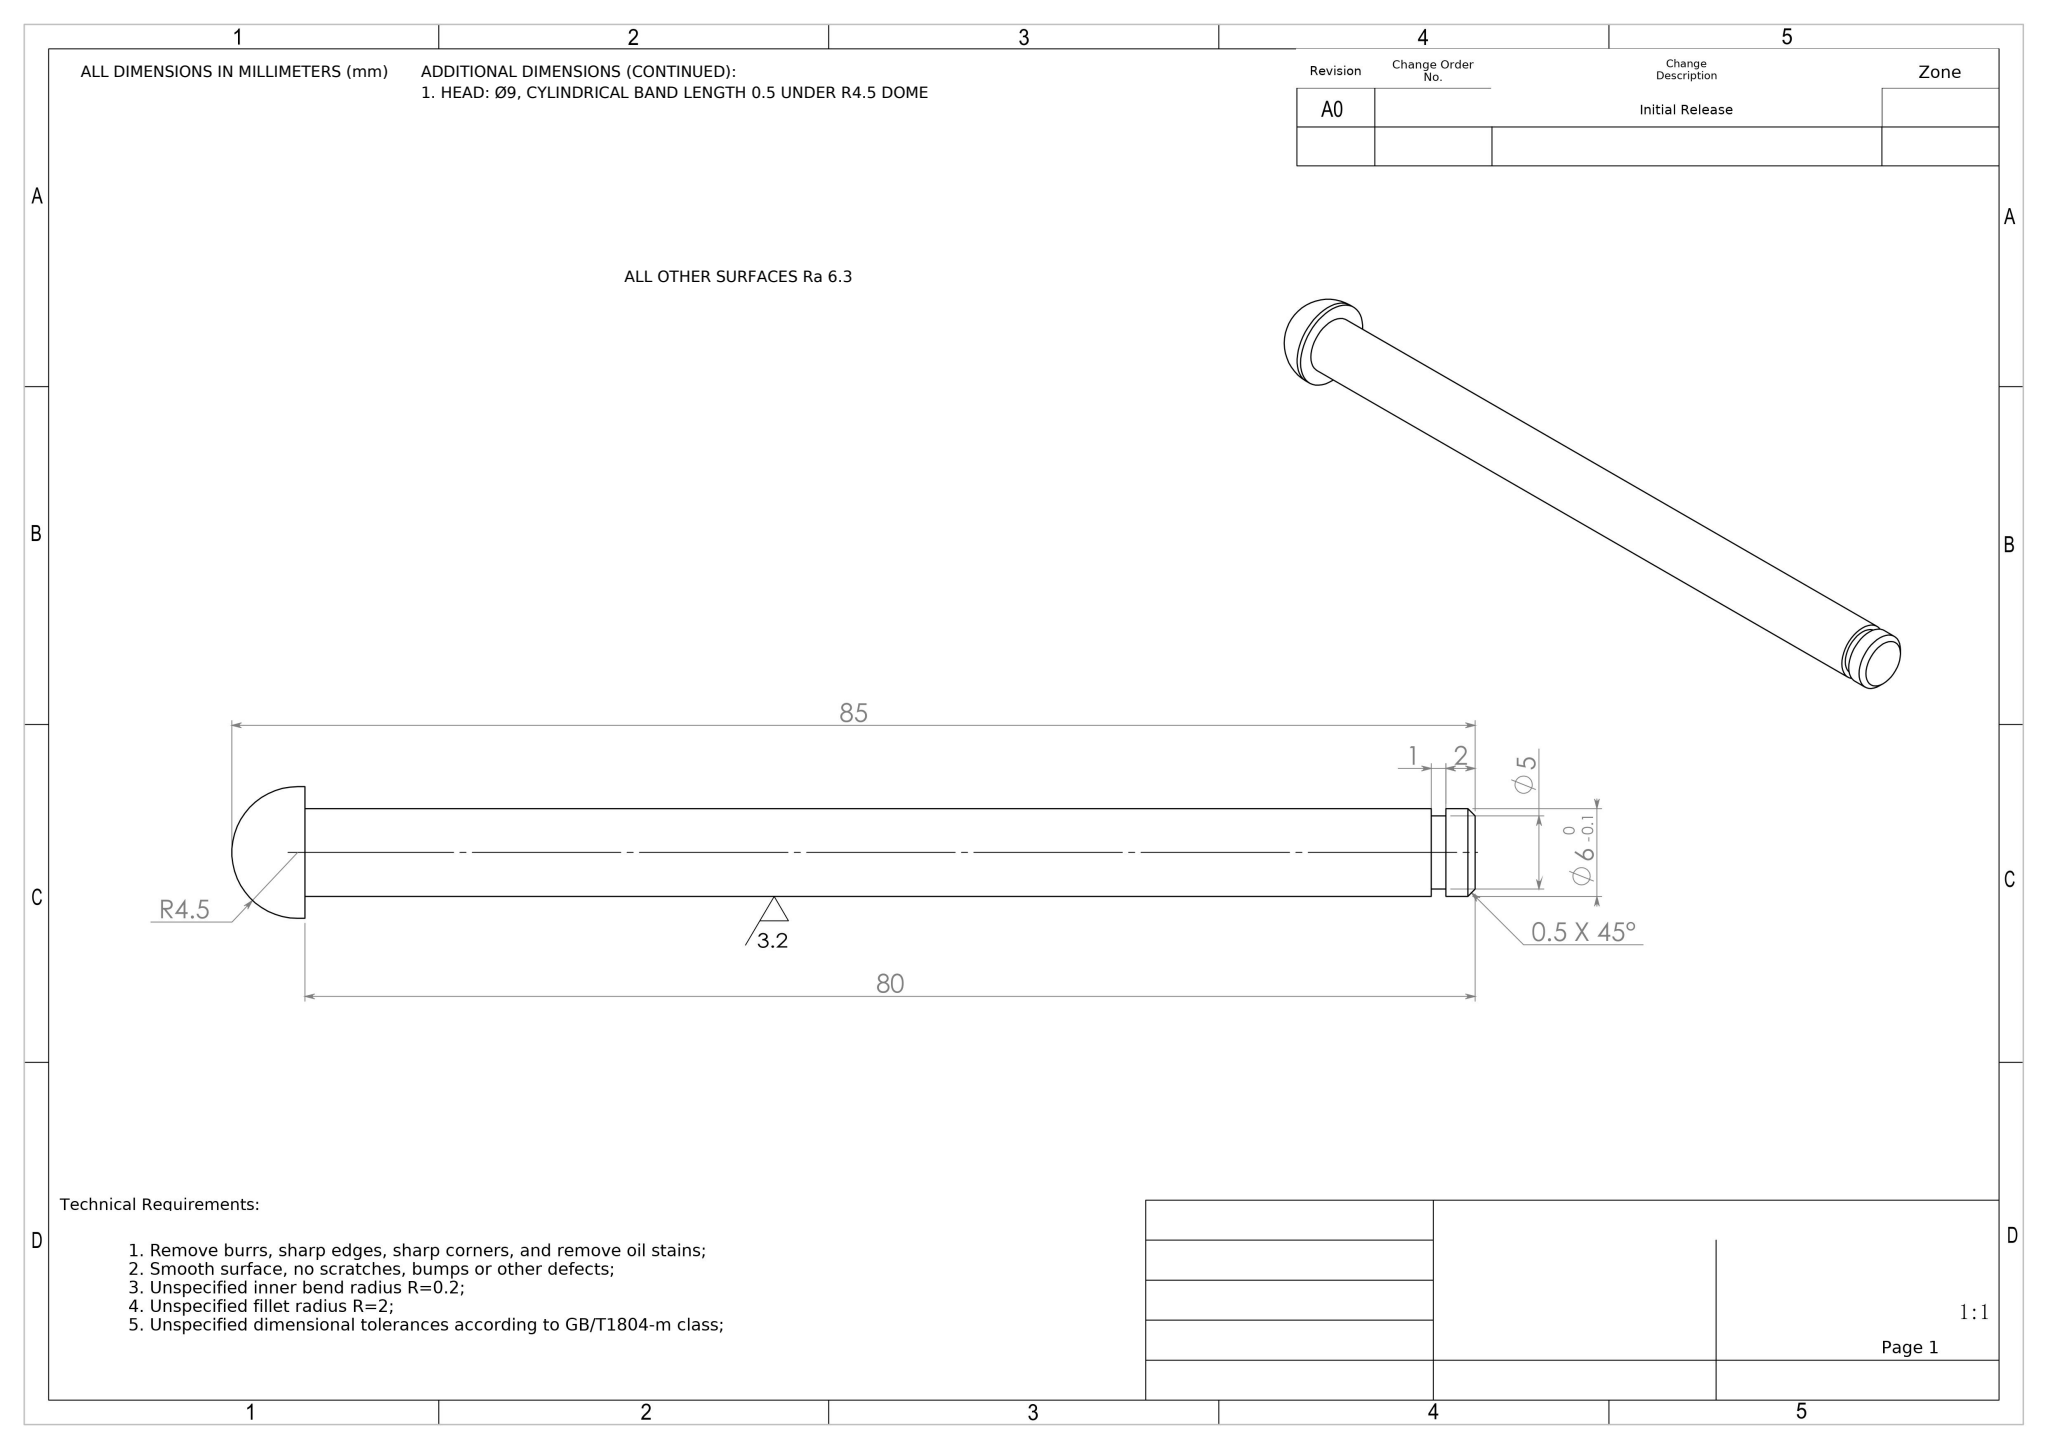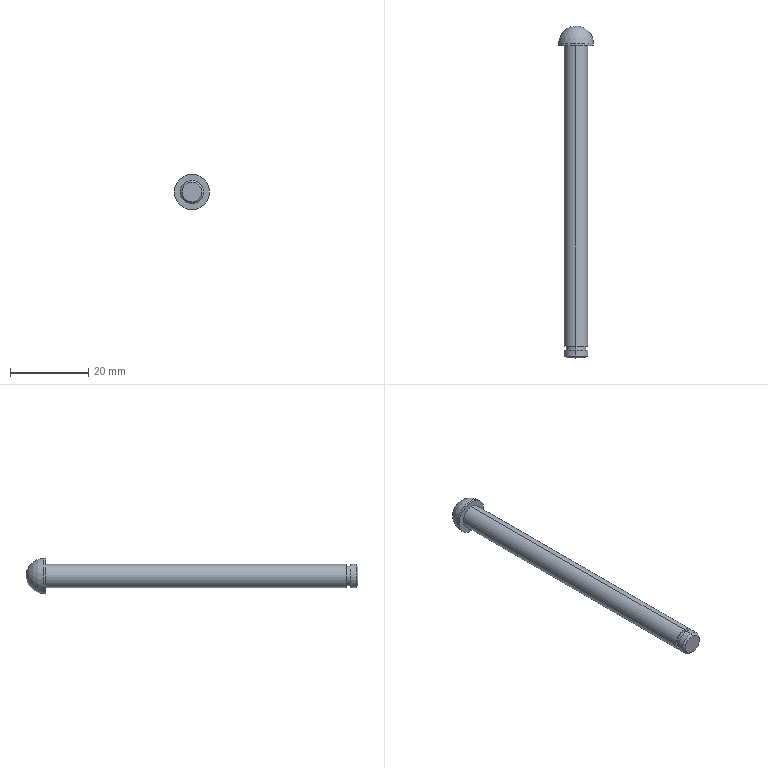Part | NX | mm | 1 solid | 15 faces | box 9 x 85 x 9 mm | volume 2474 mm3 | cylinder 8 | plane 4 | cone 2 | sphere 1 | commonest cylinder face diameters 6 x4 5 x2 9 x2
STEP:
#1=COLOUR_RGB('',0.7529,0.7529,0.7529);
#2=FILL_AREA_STYLE_COLOUR('',#1);
#3=FILL_AREA_STYLE('',(#2));
#4=SURFACE_STYLE_FILL_AREA(#3);
#5=SURFACE_SIDE_STYLE('',(#4));
#6=SURFACE_STYLE_USAGE(.BOTH.,#5);
#7=PRESENTATION_STYLE_ASSIGNMENT((#6));
#8=CARTESIAN_POINT('',(0.,2.,-3.));
#9=VERTEX_POINT('',#8);
#10=CARTESIAN_POINT('',(0.,2.,3.));
#11=VERTEX_POINT('',#10);
#12=CARTESIAN_POINT('',(0.,2.,0.));
#13=DIRECTION('',(0.,-1.,0.));
#14=DIRECTION('',(0.,0.,-1.));
#15=AXIS2_PLACEMENT_3D('',#12,#13,#14);
#16=CIRCLE('',#15,3.);
#17=EDGE_CURVE('',#9,#11,#16,.T.);
#18=ORIENTED_EDGE('',*,*,#17,.T.);
#19=CARTESIAN_POINT('',(0.,0.5,3.));
#20=VERTEX_POINT('',#19);
#21=CARTESIAN_POINT('',(0.,80.,3.));
#22=DIRECTION('',(0.,-1.,0.));
#23=VECTOR('',#22,1000.);
#24=LINE('',#21,#23);
#25=EDGE_CURVE('',#11,#20,#24,.T.);
#26=ORIENTED_EDGE('',*,*,#25,.T.);
#27=CARTESIAN_POINT('',(0.,0.5,-3.));
#28=VERTEX_POINT('',#27);
#29=CARTESIAN_POINT('',(0.,0.5,0.));
#30=DIRECTION('',(0.,1.,0.));
#31=DIRECTION('',(0.,0.,1.));
#32=AXIS2_PLACEMENT_3D('',#29,#30,#31);
#33=CIRCLE('',#32,3.);
#34=EDGE_CURVE('',#20,#28,#33,.T.);
#35=ORIENTED_EDGE('',*,*,#34,.T.);
#36=CARTESIAN_POINT('',(0.,80.,-3.));
#37=DIRECTION('',(0.,-1.,0.));
#38=VECTOR('',#37,1000.);
#39=LINE('',#36,#38);
#40=EDGE_CURVE('',#9,#28,#39,.T.);
#41=ORIENTED_EDGE('',*,*,#40,.F.);
#42=EDGE_LOOP('',(#18,#26,#35,#41));
#43=FACE_OUTER_BOUND('',#42,.T.);
#44=CARTESIAN_POINT('',(0.,80.,0.));
#45=DIRECTION('',(0.,-1.,0.));
#46=DIRECTION('',(0.,0.,-1.));
#47=AXIS2_PLACEMENT_3D('',#44,#45,#46);
#48=CYLINDRICAL_SURFACE('',#47,3.);
#49=ADVANCED_FACE('',(#43),#48,.T.);
#50=CARTESIAN_POINT('',(0.,0.,-2.5));
#51=VERTEX_POINT('',#50);
#52=CARTESIAN_POINT('',(0.,0.,2.5));
#53=VERTEX_POINT('',#52);
#54=CARTESIAN_POINT('',(0.,0.,0.));
#55=DIRECTION('',(0.,-1.,0.));
#56=DIRECTION('',(0.,0.,1.));
#57=AXIS2_PLACEMENT_3D('',#54,#55,#56);
#58=CIRCLE('',#57,2.5);
#59=EDGE_CURVE('',#51,#53,#58,.T.);
#60=ORIENTED_EDGE('',*,*,#59,.F.);
#61=CARTESIAN_POINT('',(0.,0.5,-3.));
#62=DIRECTION('',(0.,0.7071,-0.7071));
#63=VECTOR('',#62,1000.);
#64=LINE('',#61,#63);
#65=EDGE_CURVE('',#51,#28,#64,.T.);
#66=ORIENTED_EDGE('',*,*,#65,.T.);
#67=ORIENTED_EDGE('',*,*,#34,.F.);
#68=CARTESIAN_POINT('',(0.,0.5,3.));
#69=DIRECTION('',(0.,0.7071,0.7071));
#70=VECTOR('',#69,1000.);
#71=LINE('',#68,#70);
#72=EDGE_CURVE('',#53,#20,#71,.T.);
#73=ORIENTED_EDGE('',*,*,#72,.F.);
#74=EDGE_LOOP('',(#60,#66,#67,#73));
#75=FACE_OUTER_BOUND('',#74,.T.);
#76=CARTESIAN_POINT('',(0.,0.5,0.));
#77=DIRECTION('',(0.,1.,0.));
#78=DIRECTION('',(0.,0.,1.));
#79=AXIS2_PLACEMENT_3D('',#76,#77,#78);
#80=CONICAL_SURFACE('',#79,3.,0.7854);
#81=ADVANCED_FACE('',(#75),#80,.T.);
#82=CARTESIAN_POINT('',(0.,3.,-2.5));
#83=VERTEX_POINT('',#82);
#84=CARTESIAN_POINT('',(0.,3.,2.5));
#85=VERTEX_POINT('',#84);
#86=CARTESIAN_POINT('',(0.,3.,0.));
#87=DIRECTION('',(0.,-1.,0.));
#88=DIRECTION('',(0.,0.,-1.));
#89=AXIS2_PLACEMENT_3D('',#86,#87,#88);
#90=CIRCLE('',#89,2.5);
#91=EDGE_CURVE('',#83,#85,#90,.T.);
#92=ORIENTED_EDGE('',*,*,#91,.T.);
#93=CARTESIAN_POINT('',(0.,2.,2.5));
#94=VERTEX_POINT('',#93);
#95=CARTESIAN_POINT('',(0.,0.,2.5));
#96=DIRECTION('',(0.,-1.,0.));
#97=VECTOR('',#96,1000.);
#98=LINE('',#95,#97);
#99=EDGE_CURVE('',#85,#94,#98,.T.);
#100=ORIENTED_EDGE('',*,*,#99,.T.);
#101=CARTESIAN_POINT('',(0.,2.,-2.5));
#102=VERTEX_POINT('',#101);
#103=CARTESIAN_POINT('',(0.,2.,0.));
#104=DIRECTION('',(0.,-1.,0.));
#105=DIRECTION('',(0.,0.,-1.));
#106=AXIS2_PLACEMENT_3D('',#103,#104,#105);
#107=CIRCLE('',#106,2.5);
#108=EDGE_CURVE('',#102,#94,#107,.T.);
#109=ORIENTED_EDGE('',*,*,#108,.F.);
#110=CARTESIAN_POINT('',(0.,0.,-2.5));
#111=DIRECTION('',(0.,-1.,0.));
#112=VECTOR('',#111,1000.);
#113=LINE('',#110,#112);
#114=EDGE_CURVE('',#83,#102,#113,.T.);
#115=ORIENTED_EDGE('',*,*,#114,.F.);
#116=EDGE_LOOP('',(#92,#100,#109,#115));
#117=FACE_OUTER_BOUND('',#116,.T.);
#118=CARTESIAN_POINT('',(0.,0.,0.));
#119=DIRECTION('',(0.,-1.,0.));
#120=DIRECTION('',(0.,0.,-1.));
#121=AXIS2_PLACEMENT_3D('',#118,#119,#120);
#122=CYLINDRICAL_SURFACE('',#121,2.5);
#123=ADVANCED_FACE('',(#117),#122,.T.);
#124=CARTESIAN_POINT('',(0.,80.5,-4.5));
#125=VERTEX_POINT('',#124);
#126=CARTESIAN_POINT('',(0.,80.5,4.5));
#127=VERTEX_POINT('',#126);
#128=CARTESIAN_POINT('',(0.,80.5,0.));
#129=DIRECTION('',(0.,-1.,0.));
#130=DIRECTION('',(0.,0.,-1.));
#131=AXIS2_PLACEMENT_3D('',#128,#129,#130);
#132=CIRCLE('',#131,4.5);
#133=EDGE_CURVE('',#125,#127,#132,.T.);
#134=ORIENTED_EDGE('',*,*,#133,.T.);
#135=CARTESIAN_POINT('',(0.,80.,4.5));
#136=VERTEX_POINT('',#135);
#137=CARTESIAN_POINT('',(0.,85.,4.5));
#138=DIRECTION('',(0.,-1.,0.));
#139=VECTOR('',#138,1000.);
#140=LINE('',#137,#139);
#141=EDGE_CURVE('',#127,#136,#140,.T.);
#142=ORIENTED_EDGE('',*,*,#141,.T.);
#143=CARTESIAN_POINT('',(0.,80.,-4.5));
#144=VERTEX_POINT('',#143);
#145=CARTESIAN_POINT('',(0.,80.,0.));
#146=DIRECTION('',(0.,1.,0.));
#147=DIRECTION('',(0.,0.,1.));
#148=AXIS2_PLACEMENT_3D('',#145,#146,#147);
#149=CIRCLE('',#148,4.5);
#150=EDGE_CURVE('',#136,#144,#149,.T.);
#151=ORIENTED_EDGE('',*,*,#150,.T.);
#152=CARTESIAN_POINT('',(0.,85.,-4.5));
#153=DIRECTION('',(0.,-1.,0.));
#154=VECTOR('',#153,1000.);
#155=LINE('',#152,#154);
#156=EDGE_CURVE('',#125,#144,#155,.T.);
#157=ORIENTED_EDGE('',*,*,#156,.F.);
#158=EDGE_LOOP('',(#134,#142,#151,#157));
#159=FACE_OUTER_BOUND('',#158,.T.);
#160=CARTESIAN_POINT('',(0.,85.,0.));
#161=DIRECTION('',(0.,-1.,0.));
#162=DIRECTION('',(0.,0.,-1.));
#163=AXIS2_PLACEMENT_3D('',#160,#161,#162);
#164=CYLINDRICAL_SURFACE('',#163,4.5);
#165=ADVANCED_FACE('',(#159),#164,.T.);
#166=CARTESIAN_POINT('',(0.,80.,3.));
#167=VERTEX_POINT('',#166);
#168=CARTESIAN_POINT('',(0.,80.,-3.));
#169=VERTEX_POINT('',#168);
#170=CARTESIAN_POINT('',(0.,80.,0.));
#171=DIRECTION('',(0.,1.,0.));
#172=DIRECTION('',(0.,0.,1.));
#173=AXIS2_PLACEMENT_3D('',#170,#171,#172);
#174=CIRCLE('',#173,3.);
#175=EDGE_CURVE('',#167,#169,#174,.T.);
#176=ORIENTED_EDGE('',*,*,#175,.F.);
#177=CARTESIAN_POINT('',(0.,3.,3.));
#178=VERTEX_POINT('',#177);
#179=CARTESIAN_POINT('',(0.,80.,3.));
#180=DIRECTION('',(0.,-1.,0.));
#181=VECTOR('',#180,1000.);
#182=LINE('',#179,#181);
#183=EDGE_CURVE('',#167,#178,#182,.T.);
#184=ORIENTED_EDGE('',*,*,#183,.T.);
#185=CARTESIAN_POINT('',(0.,3.,-3.));
#186=VERTEX_POINT('',#185);
#187=CARTESIAN_POINT('',(0.,3.,0.));
#188=DIRECTION('',(0.,-1.,0.));
#189=DIRECTION('',(0.,0.,-1.));
#190=AXIS2_PLACEMENT_3D('',#187,#188,#189);
#191=CIRCLE('',#190,3.);
#192=EDGE_CURVE('',#186,#178,#191,.T.);
#193=ORIENTED_EDGE('',*,*,#192,.F.);
#194=CARTESIAN_POINT('',(0.,80.,-3.));
#195=DIRECTION('',(0.,-1.,0.));
#196=VECTOR('',#195,1000.);
#197=LINE('',#194,#196);
#198=EDGE_CURVE('',#169,#186,#197,.T.);
#199=ORIENTED_EDGE('',*,*,#198,.F.);
#200=EDGE_LOOP('',(#176,#184,#193,#199));
#201=FACE_OUTER_BOUND('',#200,.T.);
#202=CARTESIAN_POINT('',(0.,80.,0.));
#203=DIRECTION('',(0.,-1.,0.));
#204=DIRECTION('',(0.,0.,-1.));
#205=AXIS2_PLACEMENT_3D('',#202,#203,#204);
#206=CYLINDRICAL_SURFACE('',#205,3.);
#207=ADVANCED_FACE('',(#201),#206,.T.);
#208=ORIENTED_EDGE('',*,*,#183,.F.);
#209=CARTESIAN_POINT('',(0.,80.,0.));
#210=DIRECTION('',(0.,1.,0.));
#211=DIRECTION('',(0.,0.,1.));
#212=AXIS2_PLACEMENT_3D('',#209,#210,#211);
#213=CIRCLE('',#212,3.);
#214=EDGE_CURVE('',#169,#167,#213,.T.);
#215=ORIENTED_EDGE('',*,*,#214,.F.);
#216=ORIENTED_EDGE('',*,*,#198,.T.);
#217=CARTESIAN_POINT('',(0.,3.,0.));
#218=DIRECTION('',(0.,-1.,0.));
#219=DIRECTION('',(0.,0.,-1.));
#220=AXIS2_PLACEMENT_3D('',#217,#218,#219);
#221=CIRCLE('',#220,3.);
#222=EDGE_CURVE('',#178,#186,#221,.T.);
#223=ORIENTED_EDGE('',*,*,#222,.F.);
#224=EDGE_LOOP('',(#208,#215,#216,#223));
#225=FACE_OUTER_BOUND('',#224,.T.);
#226=CARTESIAN_POINT('',(0.,80.,0.));
#227=DIRECTION('',(0.,-1.,0.));
#228=DIRECTION('',(0.,0.,-1.));
#229=AXIS2_PLACEMENT_3D('',#226,#227,#228);
#230=CYLINDRICAL_SURFACE('',#229,3.);
#231=ADVANCED_FACE('',(#225),#230,.T.);
#232=CARTESIAN_POINT('',(0.,80.,0.));
#233=DIRECTION('',(0.,1.,0.));
#234=DIRECTION('',(0.,0.,1.));
#235=AXIS2_PLACEMENT_3D('',#232,#233,#234);
#236=CIRCLE('',#235,4.5);
#237=EDGE_CURVE('',#144,#136,#236,.T.);
#238=ORIENTED_EDGE('',*,*,#237,.F.);
#239=ORIENTED_EDGE('',*,*,#150,.F.);
#240=EDGE_LOOP('',(#238,#239));
#241=FACE_OUTER_BOUND('',#240,.T.);
#242=ORIENTED_EDGE('',*,*,#214,.T.);
#243=ORIENTED_EDGE('',*,*,#175,.T.);
#244=EDGE_LOOP('',(#242,#243));
#245=FACE_BOUND('',#244,.T.);
#246=CARTESIAN_POINT('',(0.,80.,0.));
#247=DIRECTION('',(0.,1.,0.));
#248=DIRECTION('',(0.,0.,1.));
#249=AXIS2_PLACEMENT_3D('',#246,#247,#248);
#250=PLANE('',#249);
#251=ADVANCED_FACE('',(#241,#245),#250,.F.);
#252=ORIENTED_EDGE('',*,*,#141,.F.);
#253=CARTESIAN_POINT('',(0.,80.5,0.));
#254=DIRECTION('',(0.,-1.,0.));
#255=DIRECTION('',(0.,0.,-1.));
#256=AXIS2_PLACEMENT_3D('',#253,#254,#255);
#257=CIRCLE('',#256,4.5);
#258=EDGE_CURVE('',#127,#125,#257,.T.);
#259=ORIENTED_EDGE('',*,*,#258,.T.);
#260=ORIENTED_EDGE('',*,*,#156,.T.);
#261=ORIENTED_EDGE('',*,*,#237,.T.);
#262=EDGE_LOOP('',(#252,#259,#260,#261));
#263=FACE_OUTER_BOUND('',#262,.T.);
#264=CARTESIAN_POINT('',(0.,85.,0.));
#265=DIRECTION('',(0.,-1.,0.));
#266=DIRECTION('',(0.,0.,-1.));
#267=AXIS2_PLACEMENT_3D('',#264,#265,#266);
#268=CYLINDRICAL_SURFACE('',#267,4.5);
#269=ADVANCED_FACE('',(#263),#268,.T.);
#270=ORIENTED_EDGE('',*,*,#133,.F.);
#271=ORIENTED_EDGE('',*,*,#258,.F.);
#272=EDGE_LOOP('',(#270,#271));
#273=FACE_OUTER_BOUND('',#272,.T.);
#274=CARTESIAN_POINT('',(0.,80.5,0.));
#275=DIRECTION('',(0.,1.,0.));
#276=DIRECTION('',(1.,0.,0.));
#277=AXIS2_PLACEMENT_3D('',#274,#275,#276);
#278=SPHERICAL_SURFACE('',#277,4.5);
#279=ADVANCED_FACE('',(#273),#278,.T.);
#280=ORIENTED_EDGE('',*,*,#91,.F.);
#281=CARTESIAN_POINT('',(0.,3.,0.));
#282=DIRECTION('',(0.,-1.,0.));
#283=DIRECTION('',(0.,0.,-1.));
#284=AXIS2_PLACEMENT_3D('',#281,#282,#283);
#285=CIRCLE('',#284,2.5);
#286=EDGE_CURVE('',#85,#83,#285,.T.);
#287=ORIENTED_EDGE('',*,*,#286,.F.);
#288=EDGE_LOOP('',(#280,#287));
#289=FACE_BOUND('',#288,.T.);
#290=ORIENTED_EDGE('',*,*,#192,.T.);
#291=ORIENTED_EDGE('',*,*,#222,.T.);
#292=EDGE_LOOP('',(#290,#291));
#293=FACE_OUTER_BOUND('',#292,.T.);
#294=CARTESIAN_POINT('',(3.,3.,0.));
#295=DIRECTION('',(0.,1.,0.));
#296=DIRECTION('',(0.,0.,1.));
#297=AXIS2_PLACEMENT_3D('',#294,#295,#296);
#298=PLANE('',#297);
#299=ADVANCED_FACE('',(#289,#293),#298,.F.);
#300=ORIENTED_EDGE('',*,*,#99,.F.);
#301=ORIENTED_EDGE('',*,*,#286,.T.);
#302=ORIENTED_EDGE('',*,*,#114,.T.);
#303=CARTESIAN_POINT('',(0.,2.,0.));
#304=DIRECTION('',(0.,-1.,0.));
#305=DIRECTION('',(0.,0.,-1.));
#306=AXIS2_PLACEMENT_3D('',#303,#304,#305);
#307=CIRCLE('',#306,2.5);
#308=EDGE_CURVE('',#94,#102,#307,.T.);
#309=ORIENTED_EDGE('',*,*,#308,.F.);
#310=EDGE_LOOP('',(#300,#301,#302,#309));
#311=FACE_OUTER_BOUND('',#310,.T.);
#312=CARTESIAN_POINT('',(0.,0.,0.));
#313=DIRECTION('',(0.,-1.,0.));
#314=DIRECTION('',(0.,0.,-1.));
#315=AXIS2_PLACEMENT_3D('',#312,#313,#314);
#316=CYLINDRICAL_SURFACE('',#315,2.5);
#317=ADVANCED_FACE('',(#311),#316,.T.);
#318=ORIENTED_EDGE('',*,*,#17,.F.);
#319=CARTESIAN_POINT('',(0.,2.,0.));
#320=DIRECTION('',(0.,-1.,0.));
#321=DIRECTION('',(0.,0.,-1.));
#322=AXIS2_PLACEMENT_3D('',#319,#320,#321);
#323=CIRCLE('',#322,3.);
#324=EDGE_CURVE('',#11,#9,#323,.T.);
#325=ORIENTED_EDGE('',*,*,#324,.F.);
#326=EDGE_LOOP('',(#318,#325));
#327=FACE_OUTER_BOUND('',#326,.T.);
#328=ORIENTED_EDGE('',*,*,#108,.T.);
#329=ORIENTED_EDGE('',*,*,#308,.T.);
#330=EDGE_LOOP('',(#328,#329));
#331=FACE_BOUND('',#330,.T.);
#332=CARTESIAN_POINT('',(3.,2.,0.));
#333=DIRECTION('',(0.,-1.,0.));
#334=DIRECTION('',(0.,0.,-1.));
#335=AXIS2_PLACEMENT_3D('',#332,#333,#334);
#336=PLANE('',#335);
#337=ADVANCED_FACE('',(#327,#331),#336,.F.);
#338=CARTESIAN_POINT('',(0.,0.,0.));
#339=DIRECTION('',(0.,-1.,0.));
#340=DIRECTION('',(0.,0.,1.));
#341=AXIS2_PLACEMENT_3D('',#338,#339,#340);
#342=CIRCLE('',#341,2.5);
#343=EDGE_CURVE('',#53,#51,#342,.T.);
#344=ORIENTED_EDGE('',*,*,#343,.T.);
#345=ORIENTED_EDGE('',*,*,#59,.T.);
#346=EDGE_LOOP('',(#344,#345));
#347=FACE_OUTER_BOUND('',#346,.T.);
#348=CARTESIAN_POINT('',(0.,0.,0.));
#349=DIRECTION('',(0.,1.,0.));
#350=DIRECTION('',(0.,0.,1.));
#351=AXIS2_PLACEMENT_3D('',#348,#349,#350);
#352=PLANE('',#351);
#353=ADVANCED_FACE('',(#347),#352,.F.);
#354=ORIENTED_EDGE('',*,*,#65,.F.);
#355=ORIENTED_EDGE('',*,*,#343,.F.);
#356=ORIENTED_EDGE('',*,*,#72,.T.);
#357=CARTESIAN_POINT('',(0.,0.5,0.));
#358=DIRECTION('',(0.,1.,0.));
#359=DIRECTION('',(0.,0.,1.));
#360=AXIS2_PLACEMENT_3D('',#357,#358,#359);
#361=CIRCLE('',#360,3.);
#362=EDGE_CURVE('',#28,#20,#361,.T.);
#363=ORIENTED_EDGE('',*,*,#362,.F.);
#364=EDGE_LOOP('',(#354,#355,#356,#363));
#365=FACE_OUTER_BOUND('',#364,.T.);
#366=CARTESIAN_POINT('',(0.,0.5,0.));
#367=DIRECTION('',(0.,1.,0.));
#368=DIRECTION('',(0.,0.,1.));
#369=AXIS2_PLACEMENT_3D('',#366,#367,#368);
#370=CONICAL_SURFACE('',#369,3.,0.7854);
#371=ADVANCED_FACE('',(#365),#370,.T.);
#372=ORIENTED_EDGE('',*,*,#25,.F.);
#373=ORIENTED_EDGE('',*,*,#324,.T.);
#374=ORIENTED_EDGE('',*,*,#40,.T.);
#375=ORIENTED_EDGE('',*,*,#362,.T.);
#376=EDGE_LOOP('',(#372,#373,#374,#375));
#377=FACE_OUTER_BOUND('',#376,.T.);
#378=CARTESIAN_POINT('',(0.,80.,0.));
#379=DIRECTION('',(0.,-1.,0.));
#380=DIRECTION('',(0.,0.,-1.));
#381=AXIS2_PLACEMENT_3D('',#378,#379,#380);
#382=CYLINDRICAL_SURFACE('',#381,3.);
#383=ADVANCED_FACE('',(#377),#382,.T.);
#384=CLOSED_SHELL('',(#49,#81,#123,#165,#207,#231,#251,#269,#279,#299,#317,#337,#353,#371,#383));
#385=MANIFOLD_SOLID_BREP('',#384);
#386=STYLED_ITEM('',(#7),#385);
#387=(LENGTH_UNIT()NAMED_UNIT(*)SI_UNIT(.MILLI.,.METRE.));
#388=UNCERTAINTY_MEASURE_WITH_UNIT(LENGTH_MEASURE(0.00001),#387,'','');
#389=(NAMED_UNIT(*)PLANE_ANGLE_UNIT()SI_UNIT($,.RADIAN.));
#390=(NAMED_UNIT(*)SI_UNIT($,.STERADIAN.)SOLID_ANGLE_UNIT());
#391=(GEOMETRIC_REPRESENTATION_CONTEXT(3)GLOBAL_UNCERTAINTY_ASSIGNED_CONTEXT((#388))GLOBAL_UNIT_ASSIGNED_CONTEXT((#387,#389,#390))REPRESENTATION_CONTEXT('',''));
#392=MECHANICAL_DESIGN_GEOMETRIC_PRESENTATION_REPRESENTATION('',(#386),#391);
#393=COLOUR_RGB('',0.7529,0.7529,0.7529);
#394=FILL_AREA_STYLE_COLOUR('',#393);
#395=FILL_AREA_STYLE('',(#394));
#396=SURFACE_STYLE_FILL_AREA(#395);
#397=SURFACE_SIDE_STYLE('',(#396));
#398=SURFACE_STYLE_USAGE(.BOTH.,#397);
#399=PRESENTATION_STYLE_ASSIGNMENT((#398));
#400=CARTESIAN_POINT('',(0.,0.,0.));
#401=DIRECTION('',(0.,0.,1.));
#402=DIRECTION('',(1.,0.,0.));
#403=AXIS2_PLACEMENT_3D('',#400,#401,#402);
#404=(LENGTH_UNIT()NAMED_UNIT(*)SI_UNIT(.MILLI.,.METRE.));
#405=UNCERTAINTY_MEASURE_WITH_UNIT(LENGTH_MEASURE(0.00001),#404,'','');
#406=(NAMED_UNIT(*)PLANE_ANGLE_UNIT()SI_UNIT($,.RADIAN.));
#407=(NAMED_UNIT(*)SI_UNIT($,.STERADIAN.)SOLID_ANGLE_UNIT());
#408=(GEOMETRIC_REPRESENTATION_CONTEXT(3)GLOBAL_UNCERTAINTY_ASSIGNED_CONTEXT((#405))GLOBAL_UNIT_ASSIGNED_CONTEXT((#404,#406,#407))REPRESENTATION_CONTEXT('',''));
#409=ADVANCED_BREP_SHAPE_REPRESENTATION('',(#385,#403),#408);
#410=STYLED_ITEM('',(#399),#409);
#411=(LENGTH_UNIT()NAMED_UNIT(*)SI_UNIT(.MILLI.,.METRE.));
#412=UNCERTAINTY_MEASURE_WITH_UNIT(LENGTH_MEASURE(0.00001),#411,'','');
#413=(NAMED_UNIT(*)PLANE_ANGLE_UNIT()SI_UNIT($,.RADIAN.));
#414=(NAMED_UNIT(*)SI_UNIT($,.STERADIAN.)SOLID_ANGLE_UNIT());
#415=(GEOMETRIC_REPRESENTATION_CONTEXT(3)GLOBAL_UNCERTAINTY_ASSIGNED_CONTEXT((#412))GLOBAL_UNIT_ASSIGNED_CONTEXT((#411,#413,#414))REPRESENTATION_CONTEXT('',''));
#416=MECHANICAL_DESIGN_GEOMETRIC_PRESENTATION_REPRESENTATION('',(#410),#415);
#417=PRESENTATION_LAYER_ASSIGNMENT('','',(#386));
#418=PRESENTATION_LAYER_ASSIGNMENT('','',(#410));